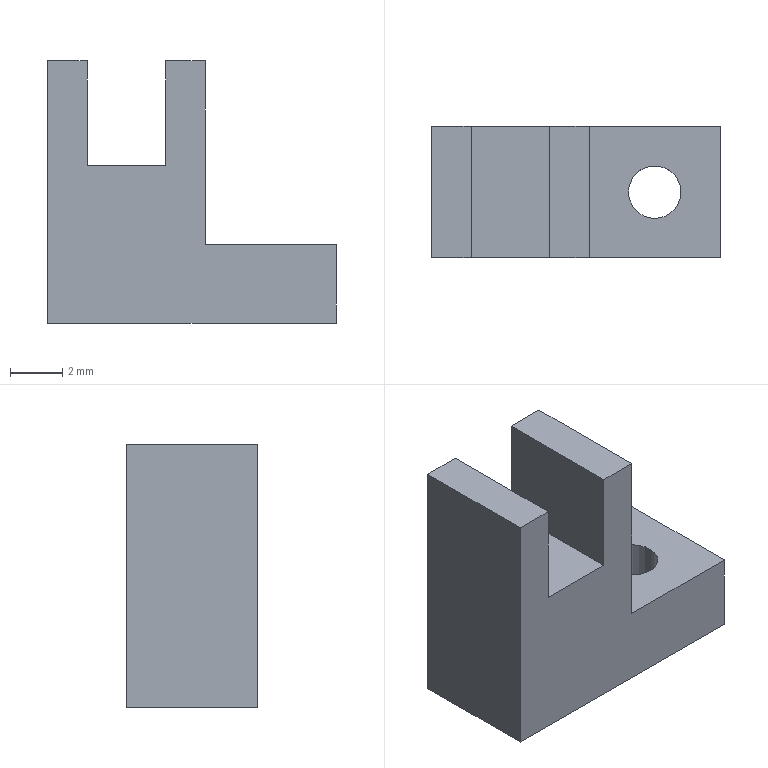Component | SolidWorks | 8-2 | 1 solid | 17 faces | box 11 x 5 x 10 mm | volume 296 mm3 | plane 13 | cylinder 4 | commonest cylinder face diameters 2 x4
build123d program:
from build123d import *

# Parameters (mm, degrees)
BOSS_EXTRUDE1_DEPTH = 5
SKETCH2_W           = 5
SKETCH2_H           = 3
BOSS_EXTRUDE2_DEPTH = 4.5
SKETCH3_W           = 5
SKETCH3_H           = 1.5
BOSS_EXTRUDE3_DEPTH = 4
SKETCH4_W           = 4
SKETCH4_H           = 5
BOSS_EXTRUDE4_DEPTH = 1.5
SKETCH5_W           = 3
SKETCH5_H           = 5
BOSS_EXTRUDE5_DEPTH = 5
SKETCH6_R           = 1
CUT_EXTRUDE1_DEPTH  = 5
SKETCH8_R           = 1
CUT_EXTRUDE8_DEPTH  = 3


with BuildPart() as part:
    # Sketch1 → Boss-Extrude1 (new body)
    with BuildSketch(Plane.XY):
        Polygon((0, 0), (-4.5, 0), (-4.5, -1.5), (1.5, -1.5), (1.5, 4.5), (-4.5, 4.5), (-4.5, 3), (0, 3), align=None)
    extrude(amount=BOSS_EXTRUDE1_DEPTH)

    # Sketch2 → Boss-Extrude2 (add)
    with BuildSketch(Plane.ZY):
        with Locations((2.5, 1.5)):
            Rectangle(SKETCH2_W, SKETCH2_H)
    extrude(amount=BOSS_EXTRUDE2_DEPTH)

    # Sketch3 → Boss-Extrude3 (add)
    with BuildSketch(Plane.ZY.offset(4.5)):
        with Locations((2.5, 3.75)):
            Rectangle(SKETCH3_W, SKETCH3_H)
    extrude(amount=BOSS_EXTRUDE3_DEPTH)

    # Sketch4 → Boss-Extrude4 (add)
    with BuildSketch(Plane.XZ.offset(1.5)):
        with Locations((-6.5, 2.5)):
            Rectangle(SKETCH4_W, SKETCH4_H)
    extrude(amount=-BOSS_EXTRUDE4_DEPTH)

    # Sketch5 → Boss-Extrude5 (add)
    with BuildSketch(Plane(origin=(0, 4.5, 0), x_dir=(1, 0, 0), z_dir=(0, 1, 0))):
        with Locations((0, -2.5)):
            Rectangle(SKETCH5_W, SKETCH5_H)
    extrude(amount=BOSS_EXTRUDE5_DEPTH)

    # Sketch6 → Cut-Extrude1 (cut)
    with BuildSketch(Plane.ZY.offset(1.5)):
        with Locations(Location((2.5, 7, 0), (0, 0, 270))):
            Circle(SKETCH6_R)
    extrude(amount=-CUT_EXTRUDE1_DEPTH, mode=Mode.SUBTRACT)

    # Sketch8 → Cut-Extrude8 (cut)
    with BuildSketch(Plane(origin=(1.5, 0, 0), x_dir=(0, 0, -1), z_dir=(1, 0, 0))):
        with Locations(Location((-2.5, 1.49, 0), (0, 0, 90))):
            Circle(SKETCH8_R)
    extrude(amount=-CUT_EXTRUDE8_DEPTH, mode=Mode.SUBTRACT)


solid = part.part

# Placed as in the assembly
solid = solid.moved(Location((64.247, 46.914, 20.438), (90, 0, -90)))
STEP:
#1=COLOUR_RGB('',0.7922,0.8196,0.9333);
#2=FILL_AREA_STYLE_COLOUR('',#1);
#3=FILL_AREA_STYLE('',(#2));
#4=SURFACE_STYLE_FILL_AREA(#3);
#5=SURFACE_SIDE_STYLE('',(#4));
#6=SURFACE_STYLE_USAGE(.BOTH.,#5);
#7=PRESENTATION_STYLE_ASSIGNMENT((#6));
#8=CARTESIAN_POINT('',(2.549,1.749,0.8637));
#9=VERTEX_POINT('',#8);
#10=CARTESIAN_POINT('',(2.627,1.749,0.8637));
#11=VERTEX_POINT('',#10);
#12=CARTESIAN_POINT('',(2.588,1.749,0.8637));
#13=DIRECTION('',(0.,-0.,-1.));
#14=DIRECTION('',(1.,0.,0.));
#15=AXIS2_PLACEMENT_3D('',#12,#13,#14);
#16=CIRCLE('',#15,0.03937);
#17=EDGE_CURVE('',#9,#11,#16,.T.);
#18=ORIENTED_EDGE('',*,*,#17,.F.);
#19=CARTESIAN_POINT('',(2.549,1.749,0.7456));
#20=VERTEX_POINT('',#19);
#21=CARTESIAN_POINT('',(2.549,1.749,0.8637));
#22=DIRECTION('',(0.,-0.,-1.));
#23=VECTOR('',#22,39.37);
#24=LINE('',#21,#23);
#25=EDGE_CURVE('',#9,#20,#24,.T.);
#26=ORIENTED_EDGE('',*,*,#25,.T.);
#27=CARTESIAN_POINT('',(2.627,1.749,0.7456));
#28=VERTEX_POINT('',#27);
#29=CARTESIAN_POINT('',(2.588,1.749,0.7456));
#30=DIRECTION('',(0.,-0.,-1.));
#31=DIRECTION('',(1.,0.,0.));
#32=AXIS2_PLACEMENT_3D('',#29,#30,#31);
#33=CIRCLE('',#32,0.03937);
#34=EDGE_CURVE('',#20,#28,#33,.T.);
#35=ORIENTED_EDGE('',*,*,#34,.T.);
#36=CARTESIAN_POINT('',(2.627,1.749,0.8637));
#37=DIRECTION('',(0.,-0.,-1.));
#38=VECTOR('',#37,39.37);
#39=LINE('',#36,#38);
#40=EDGE_CURVE('',#11,#28,#39,.T.);
#41=ORIENTED_EDGE('',*,*,#40,.F.);
#42=EDGE_LOOP('',(#18,#26,#35,#41));
#43=FACE_OUTER_BOUND('',#42,.T.);
#44=CARTESIAN_POINT('',(2.588,1.749,0.8637));
#45=DIRECTION('',(0.,-0.,-1.));
#46=DIRECTION('',(1.,0.,0.));
#47=AXIS2_PLACEMENT_3D('',#44,#45,#46);
#48=CYLINDRICAL_SURFACE('',#47,0.03937);
#49=ADVANCED_FACE('',(#43),#48,.F.);
#50=CARTESIAN_POINT('',(2.844,1.749,0.7456));
#51=VERTEX_POINT('',#50);
#52=CARTESIAN_POINT('',(2.766,1.749,0.7456));
#53=VERTEX_POINT('',#52);
#54=CARTESIAN_POINT('',(2.805,1.749,0.7456));
#55=DIRECTION('',(-0.,0.,1.));
#56=DIRECTION('',(-1.,0.,0.));
#57=AXIS2_PLACEMENT_3D('',#54,#55,#56);
#58=CIRCLE('',#57,0.03937);
#59=EDGE_CURVE('',#51,#53,#58,.T.);
#60=ORIENTED_EDGE('',*,*,#59,.F.);
#61=CARTESIAN_POINT('',(2.844,1.749,0.8637));
#62=VERTEX_POINT('',#61);
#63=CARTESIAN_POINT('',(2.844,1.749,0.6669));
#64=DIRECTION('',(0.,0.,1.));
#65=VECTOR('',#64,39.37);
#66=LINE('',#63,#65);
#67=EDGE_CURVE('',#51,#62,#66,.T.);
#68=ORIENTED_EDGE('',*,*,#67,.T.);
#69=CARTESIAN_POINT('',(2.766,1.749,0.8637));
#70=VERTEX_POINT('',#69);
#71=CARTESIAN_POINT('',(2.805,1.749,0.8637));
#72=DIRECTION('',(0.,0.,1.));
#73=DIRECTION('',(-1.,0.,0.));
#74=AXIS2_PLACEMENT_3D('',#71,#72,#73);
#75=CIRCLE('',#74,0.03937);
#76=EDGE_CURVE('',#62,#70,#75,.T.);
#77=ORIENTED_EDGE('',*,*,#76,.T.);
#78=CARTESIAN_POINT('',(2.766,1.749,0.6669));
#79=DIRECTION('',(0.,0.,1.));
#80=VECTOR('',#79,39.37);
#81=LINE('',#78,#80);
#82=EDGE_CURVE('',#53,#70,#81,.T.);
#83=ORIENTED_EDGE('',*,*,#82,.F.);
#84=EDGE_LOOP('',(#60,#68,#77,#83));
#85=FACE_OUTER_BOUND('',#84,.T.);
#86=CARTESIAN_POINT('',(2.805,1.749,0.6669));
#87=DIRECTION('',(0.,0.,1.));
#88=DIRECTION('',(-1.,0.,0.));
#89=AXIS2_PLACEMENT_3D('',#86,#87,#88);
#90=CYLINDRICAL_SURFACE('',#89,0.03937);
#91=ADVANCED_FACE('',(#85),#90,.F.);
#92=CARTESIAN_POINT('',(2.707,1.847,0.8637));
#93=VERTEX_POINT('',#92);
#94=CARTESIAN_POINT('',(2.707,1.65,0.8637));
#95=VERTEX_POINT('',#94);
#96=CARTESIAN_POINT('',(2.707,1.65,0.8637));
#97=DIRECTION('',(-0.,-1.,0.));
#98=VECTOR('',#97,39.37);
#99=LINE('',#96,#98);
#100=EDGE_CURVE('',#93,#95,#99,.T.);
#101=ORIENTED_EDGE('',*,*,#100,.F.);
#102=CARTESIAN_POINT('',(2.707,1.847,1.139));
#103=VERTEX_POINT('',#102);
#104=CARTESIAN_POINT('',(2.707,1.847,0.7456));
#105=DIRECTION('',(0.,0.,1.));
#106=VECTOR('',#105,39.37);
#107=LINE('',#104,#106);
#108=EDGE_CURVE('',#93,#103,#107,.T.);
#109=ORIENTED_EDGE('',*,*,#108,.T.);
#110=CARTESIAN_POINT('',(2.707,1.65,1.139));
#111=VERTEX_POINT('',#110);
#112=CARTESIAN_POINT('',(2.707,1.65,1.139));
#113=DIRECTION('',(0.,1.,-0.));
#114=VECTOR('',#113,39.37);
#115=LINE('',#112,#114);
#116=EDGE_CURVE('',#111,#103,#115,.T.);
#117=ORIENTED_EDGE('',*,*,#116,.F.);
#118=CARTESIAN_POINT('',(2.707,1.65,0.7456));
#119=DIRECTION('',(0.,0.,1.));
#120=VECTOR('',#119,39.37);
#121=LINE('',#118,#120);
#122=EDGE_CURVE('',#95,#111,#121,.T.);
#123=ORIENTED_EDGE('',*,*,#122,.F.);
#124=EDGE_LOOP('',(#101,#109,#117,#123));
#125=FACE_OUTER_BOUND('',#124,.T.);
#126=CARTESIAN_POINT('',(2.707,1.65,0.7456));
#127=DIRECTION('',(-1.,0.,0.));
#128=DIRECTION('',(-0.,-0.,-1.));
#129=AXIS2_PLACEMENT_3D('',#126,#127,#128);
#130=PLANE('',#129);
#131=ADVANCED_FACE('',(#125),#130,.F.);
#132=CARTESIAN_POINT('',(2.648,1.847,0.9818));
#133=VERTEX_POINT('',#132);
#134=CARTESIAN_POINT('',(2.529,1.847,0.9818));
#135=VERTEX_POINT('',#134);
#136=CARTESIAN_POINT('',(2.707,1.847,0.9818));
#137=DIRECTION('',(-1.,0.,0.));
#138=VECTOR('',#137,39.37);
#139=LINE('',#136,#138);
#140=EDGE_CURVE('',#133,#135,#139,.T.);
#141=ORIENTED_EDGE('',*,*,#140,.T.);
#142=CARTESIAN_POINT('',(2.529,1.65,0.9818));
#143=VERTEX_POINT('',#142);
#144=CARTESIAN_POINT('',(2.529,1.65,0.9818));
#145=DIRECTION('',(-0.,-1.,0.));
#146=VECTOR('',#145,39.37);
#147=LINE('',#144,#146);
#148=EDGE_CURVE('',#135,#143,#147,.T.);
#149=ORIENTED_EDGE('',*,*,#148,.T.);
#150=CARTESIAN_POINT('',(2.648,1.65,0.9818));
#151=VERTEX_POINT('',#150);
#152=CARTESIAN_POINT('',(2.529,1.65,0.9818));
#153=DIRECTION('',(-1.,0.,0.));
#154=VECTOR('',#153,39.37);
#155=LINE('',#152,#154);
#156=EDGE_CURVE('',#151,#143,#155,.T.);
#157=ORIENTED_EDGE('',*,*,#156,.F.);
#158=CARTESIAN_POINT('',(2.648,1.65,0.9818));
#159=DIRECTION('',(-0.,-1.,0.));
#160=VECTOR('',#159,39.37);
#161=LINE('',#158,#160);
#162=EDGE_CURVE('',#133,#151,#161,.T.);
#163=ORIENTED_EDGE('',*,*,#162,.F.);
#164=EDGE_LOOP('',(#141,#149,#157,#163));
#165=FACE_OUTER_BOUND('',#164,.T.);
#166=CARTESIAN_POINT('',(2.707,1.65,0.9818));
#167=DIRECTION('',(-0.,-0.,-1.));
#168=DIRECTION('',(0.,1.,-0.));
#169=AXIS2_PLACEMENT_3D('',#166,#167,#168);
#170=PLANE('',#169);
#171=ADVANCED_FACE('',(#165),#170,.F.);
#172=CARTESIAN_POINT('',(2.47,1.847,1.139));
#173=VERTEX_POINT('',#172);
#174=CARTESIAN_POINT('',(2.47,1.847,0.7456));
#175=VERTEX_POINT('',#174);
#176=CARTESIAN_POINT('',(2.47,1.847,0.7456));
#177=DIRECTION('',(-0.,-0.,-1.));
#178=VECTOR('',#177,39.37);
#179=LINE('',#176,#178);
#180=EDGE_CURVE('',#173,#175,#179,.T.);
#181=ORIENTED_EDGE('',*,*,#180,.T.);
#182=CARTESIAN_POINT('',(2.47,1.65,0.7456));
#183=VERTEX_POINT('',#182);
#184=CARTESIAN_POINT('',(2.47,1.65,0.7456));
#185=DIRECTION('',(0.,1.,-0.));
#186=VECTOR('',#185,39.37);
#187=LINE('',#184,#186);
#188=EDGE_CURVE('',#183,#175,#187,.T.);
#189=ORIENTED_EDGE('',*,*,#188,.F.);
#190=CARTESIAN_POINT('',(2.47,1.65,1.139));
#191=VERTEX_POINT('',#190);
#192=CARTESIAN_POINT('',(2.47,1.65,0.7456));
#193=DIRECTION('',(-0.,-0.,-1.));
#194=VECTOR('',#193,39.37);
#195=LINE('',#192,#194);
#196=EDGE_CURVE('',#191,#183,#195,.T.);
#197=ORIENTED_EDGE('',*,*,#196,.F.);
#198=CARTESIAN_POINT('',(2.47,1.65,1.139));
#199=DIRECTION('',(0.,1.,-0.));
#200=VECTOR('',#199,39.37);
#201=LINE('',#198,#200);
#202=EDGE_CURVE('',#191,#173,#201,.T.);
#203=ORIENTED_EDGE('',*,*,#202,.T.);
#204=EDGE_LOOP('',(#181,#189,#197,#203));
#205=FACE_OUTER_BOUND('',#204,.T.);
#206=CARTESIAN_POINT('',(2.47,1.65,0.7456));
#207=DIRECTION('',(1.,-0.,-0.));
#208=DIRECTION('',(0.,0.,1.));
#209=AXIS2_PLACEMENT_3D('',#206,#207,#208);
#210=PLANE('',#209);
#211=ADVANCED_FACE('',(#205),#210,.F.);
#212=CARTESIAN_POINT('',(2.588,1.749,0.7456));
#213=DIRECTION('',(0.,-0.,-1.));
#214=DIRECTION('',(1.,0.,0.));
#215=AXIS2_PLACEMENT_3D('',#212,#213,#214);
#216=CIRCLE('',#215,0.03937);
#217=EDGE_CURVE('',#28,#20,#216,.T.);
#218=ORIENTED_EDGE('',*,*,#217,.F.);
#219=ORIENTED_EDGE('',*,*,#34,.F.);
#220=EDGE_LOOP('',(#218,#219));
#221=FACE_BOUND('',#220,.T.);
#222=CARTESIAN_POINT('',(2.805,1.749,0.7456));
#223=DIRECTION('',(-0.,0.,1.));
#224=DIRECTION('',(-1.,0.,0.));
#225=AXIS2_PLACEMENT_3D('',#222,#223,#224);
#226=CIRCLE('',#225,0.03937);
#227=EDGE_CURVE('',#53,#51,#226,.T.);
#228=ORIENTED_EDGE('',*,*,#227,.T.);
#229=ORIENTED_EDGE('',*,*,#59,.T.);
#230=EDGE_LOOP('',(#228,#229));
#231=FACE_BOUND('',#230,.T.);
#232=CARTESIAN_POINT('',(2.903,1.847,0.7456));
#233=VERTEX_POINT('',#232);
#234=CARTESIAN_POINT('',(2.707,1.847,0.7456));
#235=DIRECTION('',(1.,-0.,0.));
#236=VECTOR('',#235,39.37);
#237=LINE('',#234,#236);
#238=EDGE_CURVE('',#175,#233,#237,.T.);
#239=ORIENTED_EDGE('',*,*,#238,.T.);
#240=CARTESIAN_POINT('',(2.903,1.65,0.7456));
#241=VERTEX_POINT('',#240);
#242=CARTESIAN_POINT('',(2.903,1.65,0.7456));
#243=DIRECTION('',(0.,1.,-0.));
#244=VECTOR('',#243,39.37);
#245=LINE('',#242,#244);
#246=EDGE_CURVE('',#241,#233,#245,.T.);
#247=ORIENTED_EDGE('',*,*,#246,.F.);
#248=CARTESIAN_POINT('',(2.707,1.65,0.7456));
#249=DIRECTION('',(1.,-0.,0.));
#250=VECTOR('',#249,39.37);
#251=LINE('',#248,#250);
#252=EDGE_CURVE('',#183,#241,#251,.T.);
#253=ORIENTED_EDGE('',*,*,#252,.F.);
#254=ORIENTED_EDGE('',*,*,#188,.T.);
#255=EDGE_LOOP('',(#239,#247,#253,#254));
#256=FACE_OUTER_BOUND('',#255,.T.);
#257=CARTESIAN_POINT('',(2.707,1.65,0.7456));
#258=DIRECTION('',(-0.,0.,1.));
#259=DIRECTION('',(-1.,0.,-0.));
#260=AXIS2_PLACEMENT_3D('',#257,#258,#259);
#261=PLANE('',#260);
#262=ADVANCED_FACE('',(#221,#231,#256),#261,.F.);
#263=ORIENTED_EDGE('',*,*,#252,.T.);
#264=CARTESIAN_POINT('',(2.903,1.65,0.8637));
#265=VERTEX_POINT('',#264);
#266=CARTESIAN_POINT('',(2.903,1.65,0.7456));
#267=DIRECTION('',(-0.,-0.,-1.));
#268=VECTOR('',#267,39.37);
#269=LINE('',#266,#268);
#270=EDGE_CURVE('',#265,#241,#269,.T.);
#271=ORIENTED_EDGE('',*,*,#270,.F.);
#272=CARTESIAN_POINT('',(2.903,1.65,0.8637));
#273=DIRECTION('',(-1.,0.,0.));
#274=VECTOR('',#273,39.37);
#275=LINE('',#272,#274);
#276=EDGE_CURVE('',#265,#95,#275,.T.);
#277=ORIENTED_EDGE('',*,*,#276,.T.);
#278=ORIENTED_EDGE('',*,*,#122,.T.);
#279=CARTESIAN_POINT('',(2.648,1.65,1.139));
#280=VERTEX_POINT('',#279);
#281=CARTESIAN_POINT('',(2.707,1.65,1.139));
#282=DIRECTION('',(1.,-0.,-0.));
#283=VECTOR('',#282,39.37);
#284=LINE('',#281,#283);
#285=EDGE_CURVE('',#280,#111,#284,.T.);
#286=ORIENTED_EDGE('',*,*,#285,.F.);
#287=CARTESIAN_POINT('',(2.648,1.65,1.139));
#288=DIRECTION('',(-0.,-0.,-1.));
#289=VECTOR('',#288,39.37);
#290=LINE('',#287,#289);
#291=EDGE_CURVE('',#280,#151,#290,.T.);
#292=ORIENTED_EDGE('',*,*,#291,.T.);
#293=ORIENTED_EDGE('',*,*,#156,.T.);
#294=CARTESIAN_POINT('',(2.529,1.65,1.139));
#295=VERTEX_POINT('',#294);
#296=CARTESIAN_POINT('',(2.529,1.65,0.9818));
#297=DIRECTION('',(0.,0.,1.));
#298=VECTOR('',#297,39.37);
#299=LINE('',#296,#298);
#300=EDGE_CURVE('',#143,#295,#299,.T.);
#301=ORIENTED_EDGE('',*,*,#300,.T.);
#302=CARTESIAN_POINT('',(2.529,1.65,1.139));
#303=DIRECTION('',(-1.,0.,0.));
#304=VECTOR('',#303,39.37);
#305=LINE('',#302,#304);
#306=EDGE_CURVE('',#295,#191,#305,.T.);
#307=ORIENTED_EDGE('',*,*,#306,.T.);
#308=ORIENTED_EDGE('',*,*,#196,.T.);
#309=EDGE_LOOP('',(#263,#271,#277,#278,#286,#292,#293,#301,#307,#308));
#310=FACE_OUTER_BOUND('',#309,.T.);
#311=CARTESIAN_POINT('',(2.529,1.65,0.8047));
#312=DIRECTION('',(0.,1.,-0.));
#313=DIRECTION('',(0.,0.,1.));
#314=AXIS2_PLACEMENT_3D('',#311,#312,#313);
#315=PLANE('',#314);
#316=ADVANCED_FACE('',(#310),#315,.F.);
#317=ORIENTED_EDGE('',*,*,#180,.F.);
#318=CARTESIAN_POINT('',(2.529,1.847,1.139));
#319=VERTEX_POINT('',#318);
#320=CARTESIAN_POINT('',(2.529,1.847,1.139));
#321=DIRECTION('',(-1.,0.,0.));
#322=VECTOR('',#321,39.37);
#323=LINE('',#320,#322);
#324=EDGE_CURVE('',#319,#173,#323,.T.);
#325=ORIENTED_EDGE('',*,*,#324,.F.);
#326=CARTESIAN_POINT('',(2.529,1.847,0.9818));
#327=DIRECTION('',(-0.,-0.,-1.));
#328=VECTOR('',#327,39.37);
#329=LINE('',#326,#328);
#330=EDGE_CURVE('',#319,#135,#329,.T.);
#331=ORIENTED_EDGE('',*,*,#330,.T.);
#332=ORIENTED_EDGE('',*,*,#140,.F.);
#333=CARTESIAN_POINT('',(2.648,1.847,1.139));
#334=VERTEX_POINT('',#333);
#335=CARTESIAN_POINT('',(2.648,1.847,1.139));
#336=DIRECTION('',(-0.,-0.,-1.));
#337=VECTOR('',#336,39.37);
#338=LINE('',#335,#337);
#339=EDGE_CURVE('',#334,#133,#338,.T.);
#340=ORIENTED_EDGE('',*,*,#339,.F.);
#341=CARTESIAN_POINT('',(2.707,1.847,1.139));
#342=DIRECTION('',(-1.,0.,0.));
#343=VECTOR('',#342,39.37);
#344=LINE('',#341,#343);
#345=EDGE_CURVE('',#103,#334,#344,.T.);
#346=ORIENTED_EDGE('',*,*,#345,.F.);
#347=ORIENTED_EDGE('',*,*,#108,.F.);
#348=CARTESIAN_POINT('',(2.903,1.847,0.8637));
#349=VERTEX_POINT('',#348);
#350=CARTESIAN_POINT('',(2.903,1.847,0.8637));
#351=DIRECTION('',(-1.,0.,0.));
#352=VECTOR('',#351,39.37);
#353=LINE('',#350,#352);
#354=EDGE_CURVE('',#349,#93,#353,.T.);
#355=ORIENTED_EDGE('',*,*,#354,.F.);
#356=CARTESIAN_POINT('',(2.903,1.847,0.7456));
#357=DIRECTION('',(0.,0.,1.));
#358=VECTOR('',#357,39.37);
#359=LINE('',#356,#358);
#360=EDGE_CURVE('',#233,#349,#359,.T.);
#361=ORIENTED_EDGE('',*,*,#360,.F.);
#362=ORIENTED_EDGE('',*,*,#238,.F.);
#363=EDGE_LOOP('',(#317,#325,#331,#332,#340,#346,#347,#355,#361,#362));
#364=FACE_OUTER_BOUND('',#363,.T.);
#365=CARTESIAN_POINT('',(2.529,1.847,0.8047));
#366=DIRECTION('',(0.,1.,-0.));
#367=DIRECTION('',(0.,0.,1.));
#368=AXIS2_PLACEMENT_3D('',#365,#366,#367);
#369=PLANE('',#368);
#370=ADVANCED_FACE('',(#364),#369,.T.);
#371=ORIENTED_EDGE('',*,*,#162,.T.);
#372=ORIENTED_EDGE('',*,*,#291,.F.);
#373=CARTESIAN_POINT('',(2.648,1.65,1.139));
#374=DIRECTION('',(-0.,-1.,0.));
#375=VECTOR('',#374,39.37);
#376=LINE('',#373,#375);
#377=EDGE_CURVE('',#334,#280,#376,.T.);
#378=ORIENTED_EDGE('',*,*,#377,.F.);
#379=ORIENTED_EDGE('',*,*,#339,.T.);
#380=EDGE_LOOP('',(#371,#372,#378,#379));
#381=FACE_OUTER_BOUND('',#380,.T.);
#382=CARTESIAN_POINT('',(2.648,1.65,1.139));
#383=DIRECTION('',(1.,-0.,-0.));
#384=DIRECTION('',(-0.,-1.,0.));
#385=AXIS2_PLACEMENT_3D('',#382,#383,#384);
#386=PLANE('',#385);
#387=ADVANCED_FACE('',(#381),#386,.F.);
#388=ORIENTED_EDGE('',*,*,#285,.T.);
#389=ORIENTED_EDGE('',*,*,#116,.T.);
#390=ORIENTED_EDGE('',*,*,#345,.T.);
#391=ORIENTED_EDGE('',*,*,#377,.T.);
#392=EDGE_LOOP('',(#388,#389,#390,#391));
#393=FACE_OUTER_BOUND('',#392,.T.);
#394=CARTESIAN_POINT('',(2.529,1.847,1.139));
#395=DIRECTION('',(-0.,-0.,-1.));
#396=DIRECTION('',(0.,1.,-0.));
#397=AXIS2_PLACEMENT_3D('',#394,#395,#396);
#398=PLANE('',#397);
#399=ADVANCED_FACE('',(#393),#398,.F.);
#400=ORIENTED_EDGE('',*,*,#202,.F.);
#401=ORIENTED_EDGE('',*,*,#306,.F.);
#402=CARTESIAN_POINT('',(2.529,1.65,1.139));
#403=DIRECTION('',(0.,1.,-0.));
#404=VECTOR('',#403,39.37);
#405=LINE('',#402,#404);
#406=EDGE_CURVE('',#295,#319,#405,.T.);
#407=ORIENTED_EDGE('',*,*,#406,.T.);
#408=ORIENTED_EDGE('',*,*,#324,.T.);
#409=EDGE_LOOP('',(#400,#401,#407,#408));
#410=FACE_OUTER_BOUND('',#409,.T.);
#411=CARTESIAN_POINT('',(2.529,1.65,1.139));
#412=DIRECTION('',(0.,0.,1.));
#413=DIRECTION('',(-1.,0.,0.));
#414=AXIS2_PLACEMENT_3D('',#411,#412,#413);
#415=PLANE('',#414);
#416=ADVANCED_FACE('',(#410),#415,.T.);
#417=ORIENTED_EDGE('',*,*,#148,.F.);
#418=ORIENTED_EDGE('',*,*,#330,.F.);
#419=ORIENTED_EDGE('',*,*,#406,.F.);
#420=ORIENTED_EDGE('',*,*,#300,.F.);
#421=EDGE_LOOP('',(#417,#418,#419,#420));
#422=FACE_OUTER_BOUND('',#421,.T.);
#423=CARTESIAN_POINT('',(2.529,1.847,0.8047));
#424=DIRECTION('',(1.,-0.,-0.));
#425=DIRECTION('',(-0.,-1.,0.));
#426=AXIS2_PLACEMENT_3D('',#423,#424,#425);
#427=PLANE('',#426);
#428=ADVANCED_FACE('',(#422),#427,.T.);
#429=CARTESIAN_POINT('',(2.805,1.749,0.8637));
#430=DIRECTION('',(0.,0.,1.));
#431=DIRECTION('',(-1.,0.,0.));
#432=AXIS2_PLACEMENT_3D('',#429,#430,#431);
#433=CIRCLE('',#432,0.03937);
#434=EDGE_CURVE('',#70,#62,#433,.T.);
#435=ORIENTED_EDGE('',*,*,#434,.F.);
#436=ORIENTED_EDGE('',*,*,#76,.F.);
#437=EDGE_LOOP('',(#435,#436));
#438=FACE_BOUND('',#437,.T.);
#439=ORIENTED_EDGE('',*,*,#100,.T.);
#440=ORIENTED_EDGE('',*,*,#276,.F.);
#441=CARTESIAN_POINT('',(2.903,1.65,0.8637));
#442=DIRECTION('',(-0.,-1.,0.));
#443=VECTOR('',#442,39.37);
#444=LINE('',#441,#443);
#445=EDGE_CURVE('',#349,#265,#444,.T.);
#446=ORIENTED_EDGE('',*,*,#445,.F.);
#447=ORIENTED_EDGE('',*,*,#354,.T.);
#448=EDGE_LOOP('',(#439,#440,#446,#447));
#449=FACE_OUTER_BOUND('',#448,.T.);
#450=CARTESIAN_POINT('',(2.903,1.65,0.8637));
#451=DIRECTION('',(-0.,-0.,-1.));
#452=DIRECTION('',(1.,-0.,-0.));
#453=AXIS2_PLACEMENT_3D('',#450,#451,#452);
#454=PLANE('',#453);
#455=ADVANCED_FACE('',(#438,#449),#454,.F.);
#456=ORIENTED_EDGE('',*,*,#246,.T.);
#457=ORIENTED_EDGE('',*,*,#360,.T.);
#458=ORIENTED_EDGE('',*,*,#445,.T.);
#459=ORIENTED_EDGE('',*,*,#270,.T.);
#460=EDGE_LOOP('',(#456,#457,#458,#459));
#461=FACE_OUTER_BOUND('',#460,.T.);
#462=CARTESIAN_POINT('',(2.903,1.847,0.8047));
#463=DIRECTION('',(1.,-0.,-0.));
#464=DIRECTION('',(0.,0.,1.));
#465=AXIS2_PLACEMENT_3D('',#462,#463,#464);
#466=PLANE('',#465);
#467=ADVANCED_FACE('',(#461),#466,.T.);
#468=ORIENTED_EDGE('',*,*,#67,.F.);
#469=ORIENTED_EDGE('',*,*,#227,.F.);
#470=ORIENTED_EDGE('',*,*,#82,.T.);
#471=ORIENTED_EDGE('',*,*,#434,.T.);
#472=EDGE_LOOP('',(#468,#469,#470,#471));
#473=FACE_OUTER_BOUND('',#472,.T.);
#474=CARTESIAN_POINT('',(2.805,1.749,0.6669));
#475=DIRECTION('',(0.,0.,1.));
#476=DIRECTION('',(-1.,0.,0.));
#477=AXIS2_PLACEMENT_3D('',#474,#475,#476);
#478=CYLINDRICAL_SURFACE('',#477,0.03937);
#479=ADVANCED_FACE('',(#473),#478,.F.);
#480=ORIENTED_EDGE('',*,*,#25,.F.);
#481=CARTESIAN_POINT('',(2.588,1.749,0.8637));
#482=DIRECTION('',(0.,-0.,-1.));
#483=DIRECTION('',(1.,0.,0.));
#484=AXIS2_PLACEMENT_3D('',#481,#482,#483);
#485=CIRCLE('',#484,0.03937);
#486=EDGE_CURVE('',#11,#9,#485,.T.);
#487=ORIENTED_EDGE('',*,*,#486,.F.);
#488=ORIENTED_EDGE('',*,*,#40,.T.);
#489=ORIENTED_EDGE('',*,*,#217,.T.);
#490=EDGE_LOOP('',(#480,#487,#488,#489));
#491=FACE_OUTER_BOUND('',#490,.T.);
#492=CARTESIAN_POINT('',(2.588,1.749,0.8637));
#493=DIRECTION('',(0.,-0.,-1.));
#494=DIRECTION('',(1.,0.,0.));
#495=AXIS2_PLACEMENT_3D('',#492,#493,#494);
#496=CYLINDRICAL_SURFACE('',#495,0.03937);
#497=ADVANCED_FACE('',(#491),#496,.F.);
#498=ORIENTED_EDGE('',*,*,#486,.T.);
#499=ORIENTED_EDGE('',*,*,#17,.T.);
#500=EDGE_LOOP('',(#498,#499));
#501=FACE_OUTER_BOUND('',#500,.T.);
#502=CARTESIAN_POINT('',(2.588,1.749,0.8637));
#503=DIRECTION('',(0.,-0.,-1.));
#504=DIRECTION('',(1.,-0.,0.));
#505=AXIS2_PLACEMENT_3D('',#502,#503,#504);
#506=PLANE('',#505);
#507=ADVANCED_FACE('',(#501),#506,.T.);
#508=CLOSED_SHELL('',(#49,#91,#131,#171,#211,#262,#316,#370,#387,#399,#416,#428,#455,#467,#479,#497,#507));
#509=MANIFOLD_SOLID_BREP('',#508);
#510=STYLED_ITEM('',(#7),#509);
#511=(LENGTH_UNIT()NAMED_UNIT(*)SI_UNIT($,.METRE.));
#512=LENGTH_MEASURE_WITH_UNIT(LENGTH_MEASURE(0.0254),#511);
#513=DIMENSIONAL_EXPONENTS(1.,0.,0.,0.,0.,0.,0.);
#514=(CONVERSION_BASED_UNIT('',#512)LENGTH_UNIT()NAMED_UNIT(#513));
#515=UNCERTAINTY_MEASURE_WITH_UNIT(LENGTH_MEASURE(0.00001),#514,'','');
#516=(NAMED_UNIT(*)PLANE_ANGLE_UNIT()SI_UNIT($,.RADIAN.));
#517=(NAMED_UNIT(*)SI_UNIT($,.STERADIAN.)SOLID_ANGLE_UNIT());
#518=(GEOMETRIC_REPRESENTATION_CONTEXT(3)GLOBAL_UNCERTAINTY_ASSIGNED_CONTEXT((#515))GLOBAL_UNIT_ASSIGNED_CONTEXT((#514,#516,#517))REPRESENTATION_CONTEXT('',''));
#519=MECHANICAL_DESIGN_GEOMETRIC_PRESENTATION_REPRESENTATION('',(#510),#518);
#520=CARTESIAN_POINT('',(0.,0.,0.));
#521=DIRECTION('',(0.,0.,1.));
#522=DIRECTION('',(1.,0.,0.));
#523=AXIS2_PLACEMENT_3D('',#520,#521,#522);
#524=(LENGTH_UNIT()NAMED_UNIT(*)SI_UNIT($,.METRE.));
#525=LENGTH_MEASURE_WITH_UNIT(LENGTH_MEASURE(0.0254),#524);
#526=DIMENSIONAL_EXPONENTS(1.,0.,0.,0.,0.,0.,0.);
#527=(CONVERSION_BASED_UNIT('',#525)LENGTH_UNIT()NAMED_UNIT(#526));
#528=UNCERTAINTY_MEASURE_WITH_UNIT(LENGTH_MEASURE(0.00001),#527,'','');
#529=(NAMED_UNIT(*)PLANE_ANGLE_UNIT()SI_UNIT($,.RADIAN.));
#530=(NAMED_UNIT(*)SI_UNIT($,.STERADIAN.)SOLID_ANGLE_UNIT());
#531=(GEOMETRIC_REPRESENTATION_CONTEXT(3)GLOBAL_UNCERTAINTY_ASSIGNED_CONTEXT((#528))GLOBAL_UNIT_ASSIGNED_CONTEXT((#527,#529,#530))REPRESENTATION_CONTEXT('',''));
#532=ADVANCED_BREP_SHAPE_REPRESENTATION('',(#509,#523),#531);
#533=PRESENTATION_LAYER_ASSIGNMENT('','',(#510));